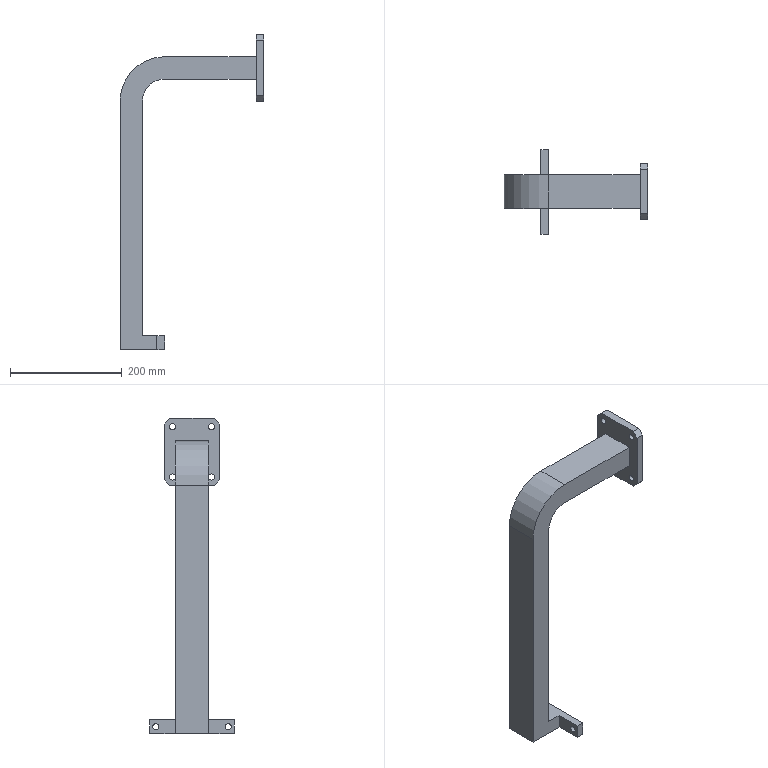Component | NX | GLUE_ARM | 1 solid | 31 faces | volume 1937212 mm3 | plane 23 | cylinder 8 | commonest cylinder face diameters 11 x6 80 x1 160 x1